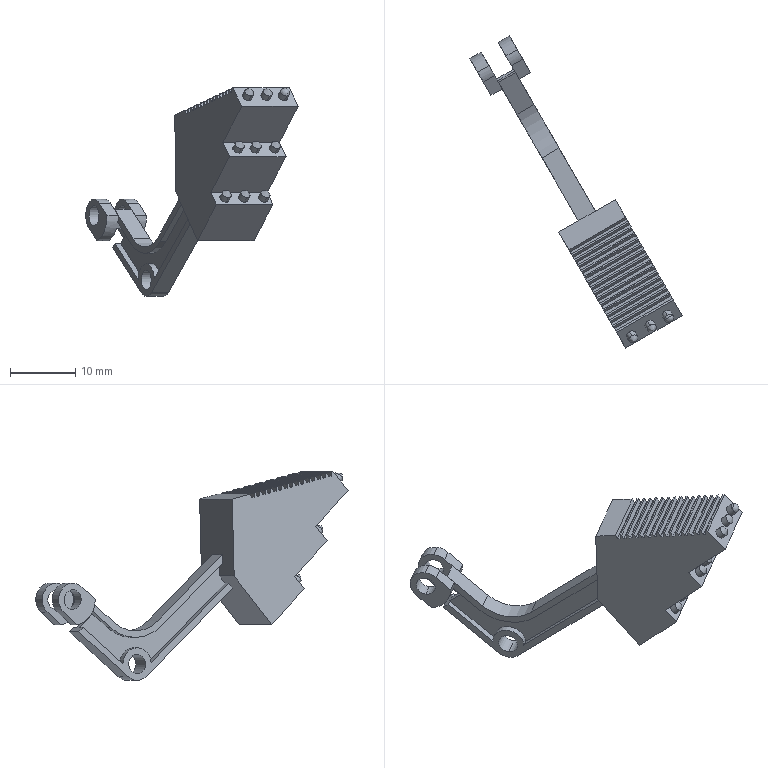Component | SolidWorks | Jaw2-3 | 1 solid | 148 faces | volume 3093 mm3 | plane 99 | cylinder 39 | spline 8 | sphere 2 | commonest cylinder face diameters 1.5 x18 5 x8 3 x6 14 x3 8 x2 6 x1 12 x1